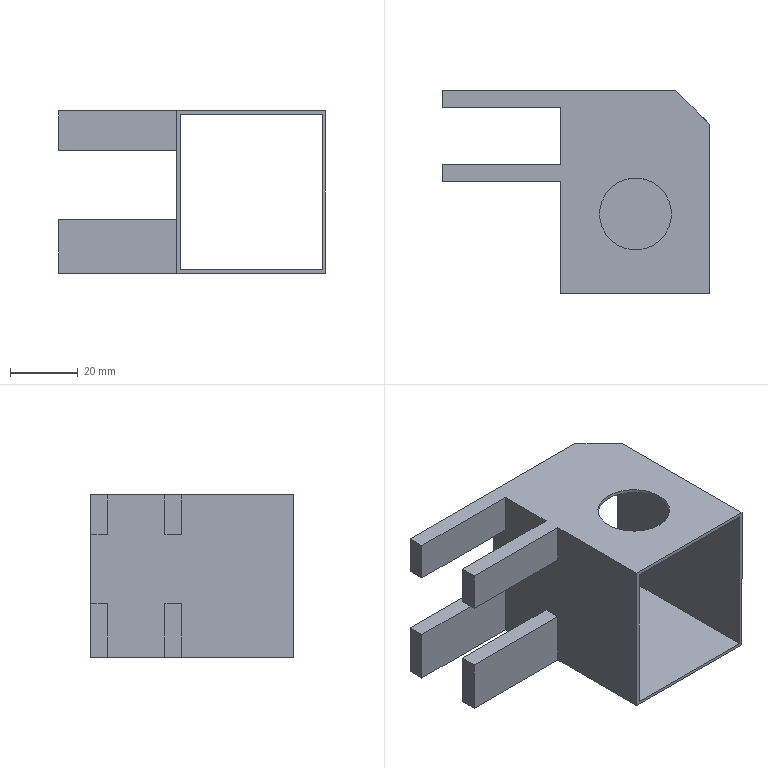Component | SolidWorks | ProtectiveCover-1 | 1 solid | 27 faces | box 79 x 60 x 48 mm | volume 19454 mm3 | plane 25 | cylinder 2 | commonest cylinder face diameters 21.247 x2
STEP:
#1=CARTESIAN_POINT('',(-2.546,-0.8182,36.42));
#2=VERTEX_POINT('',#1);
#3=CARTESIAN_POINT('',(-2.546,-1.655,36.42));
#4=VERTEX_POINT('',#3);
#5=CARTESIAN_POINT('',(-2.546,-1.236,36.42));
#6=DIRECTION('',(-0.,0.,-1.));
#7=DIRECTION('',(0.,-1.,0.));
#8=AXIS2_PLACEMENT_3D('',#5,#6,#7);
#9=CIRCLE('',#8,0.4182);
#10=EDGE_CURVE('',#2,#4,#9,.T.);
#11=ORIENTED_EDGE('',*,*,#10,.T.);
#12=CARTESIAN_POINT('',(-2.546,-1.655,36.459));
#13=VERTEX_POINT('',#12);
#14=CARTESIAN_POINT('',(-2.546,-1.655,35.107));
#15=DIRECTION('',(0.,-0.,1.));
#16=VECTOR('',#15,39.37);
#17=LINE('',#14,#16);
#18=EDGE_CURVE('',#4,#13,#17,.T.);
#19=ORIENTED_EDGE('',*,*,#18,.T.);
#20=CARTESIAN_POINT('',(-2.546,-0.8182,36.459));
#21=VERTEX_POINT('',#20);
#22=CARTESIAN_POINT('',(-2.546,-1.236,36.459));
#23=DIRECTION('',(0.,-0.,1.));
#24=DIRECTION('',(0.,1.,0.));
#25=AXIS2_PLACEMENT_3D('',#22,#23,#24);
#26=CIRCLE('',#25,0.4182);
#27=EDGE_CURVE('',#13,#21,#26,.T.);
#28=ORIENTED_EDGE('',*,*,#27,.T.);
#29=CARTESIAN_POINT('',(-2.546,-0.8182,35.107));
#30=DIRECTION('',(0.,-0.,1.));
#31=VECTOR('',#30,39.37);
#32=LINE('',#29,#31);
#33=EDGE_CURVE('',#2,#21,#32,.T.);
#34=ORIENTED_EDGE('',*,*,#33,.F.);
#35=EDGE_LOOP('',(#11,#19,#28,#34));
#36=FACE_OUTER_BOUND('',#35,.T.);
#37=CARTESIAN_POINT('',(-2.546,-1.236,35.107));
#38=DIRECTION('',(0.,-0.,1.));
#39=DIRECTION('',(0.,1.,0.));
#40=AXIS2_PLACEMENT_3D('',#37,#38,#39);
#41=CYLINDRICAL_SURFACE('',#40,0.4182);
#42=ADVANCED_FACE('',(#36),#41,.F.);
#43=CARTESIAN_POINT('',(-3.417,-0.8584,34.569));
#44=VERTEX_POINT('',#43);
#45=CARTESIAN_POINT('',(-3.417,-0.8584,35.189));
#46=VERTEX_POINT('',#45);
#47=CARTESIAN_POINT('',(-3.417,-0.8584,35.189));
#48=DIRECTION('',(0.,-0.,1.));
#49=VECTOR('',#48,39.37);
#50=LINE('',#47,#49);
#51=EDGE_CURVE('',#44,#46,#50,.T.);
#52=ORIENTED_EDGE('',*,*,#51,.F.);
#53=CARTESIAN_POINT('',(-3.417,-2.16,34.569));
#54=VERTEX_POINT('',#53);
#55=CARTESIAN_POINT('',(-3.417,-2.16,34.569));
#56=DIRECTION('',(0.,1.,0.));
#57=VECTOR('',#56,39.37);
#58=LINE('',#55,#57);
#59=EDGE_CURVE('',#54,#44,#58,.T.);
#60=ORIENTED_EDGE('',*,*,#59,.F.);
#61=CARTESIAN_POINT('',(-3.417,-2.16,36.459));
#62=VERTEX_POINT('',#61);
#63=CARTESIAN_POINT('',(-3.417,-2.16,36.459));
#64=DIRECTION('',(-0.,0.,-1.));
#65=VECTOR('',#64,39.37);
#66=LINE('',#63,#65);
#67=EDGE_CURVE('',#62,#54,#66,.T.);
#68=ORIENTED_EDGE('',*,*,#67,.F.);
#69=CARTESIAN_POINT('',(-3.417,-0.8584,36.459));
#70=VERTEX_POINT('',#69);
#71=CARTESIAN_POINT('',(-3.417,-2.16,36.459));
#72=DIRECTION('',(0.,1.,0.));
#73=VECTOR('',#72,39.37);
#74=LINE('',#71,#73);
#75=EDGE_CURVE('',#62,#70,#74,.T.);
#76=ORIENTED_EDGE('',*,*,#75,.T.);
#77=CARTESIAN_POINT('',(-3.417,-0.8584,35.997));
#78=VERTEX_POINT('',#77);
#79=CARTESIAN_POINT('',(-3.417,-0.8584,36.459));
#80=DIRECTION('',(0.,-0.,1.));
#81=VECTOR('',#80,39.37);
#82=LINE('',#79,#81);
#83=EDGE_CURVE('',#78,#70,#82,.T.);
#84=ORIENTED_EDGE('',*,*,#83,.F.);
#85=CARTESIAN_POINT('',(-3.417,-0.663,35.997));
#86=VERTEX_POINT('',#85);
#87=CARTESIAN_POINT('',(-3.417,-0.8584,35.997));
#88=DIRECTION('',(-0.,-1.,-0.));
#89=VECTOR('',#88,39.37);
#90=LINE('',#87,#89);
#91=EDGE_CURVE('',#86,#78,#90,.T.);
#92=ORIENTED_EDGE('',*,*,#91,.F.);
#93=CARTESIAN_POINT('',(-3.417,-0.663,36.459));
#94=VERTEX_POINT('',#93);
#95=CARTESIAN_POINT('',(-3.417,-0.663,36.459));
#96=DIRECTION('',(-0.,0.,-1.));
#97=VECTOR('',#96,39.37);
#98=LINE('',#95,#97);
#99=EDGE_CURVE('',#94,#86,#98,.T.);
#100=ORIENTED_EDGE('',*,*,#99,.F.);
#101=CARTESIAN_POINT('',(-3.417,0.006968,36.459));
#102=VERTEX_POINT('',#101);
#103=CARTESIAN_POINT('',(-3.417,-2.16,36.459));
#104=DIRECTION('',(0.,1.,0.));
#105=VECTOR('',#104,39.37);
#106=LINE('',#103,#105);
#107=EDGE_CURVE('',#94,#102,#106,.T.);
#108=ORIENTED_EDGE('',*,*,#107,.T.);
#109=CARTESIAN_POINT('',(-3.417,0.006968,35.997));
#110=VERTEX_POINT('',#109);
#111=CARTESIAN_POINT('',(-3.417,0.006968,36.459));
#112=DIRECTION('',(0.,-0.,1.));
#113=VECTOR('',#112,39.37);
#114=LINE('',#111,#113);
#115=EDGE_CURVE('',#110,#102,#114,.T.);
#116=ORIENTED_EDGE('',*,*,#115,.F.);
#117=CARTESIAN_POINT('',(-3.417,0.2024,35.997));
#118=VERTEX_POINT('',#117);
#119=CARTESIAN_POINT('',(-3.417,0.006968,35.997));
#120=DIRECTION('',(-0.,-1.,-0.));
#121=VECTOR('',#120,39.37);
#122=LINE('',#119,#121);
#123=EDGE_CURVE('',#118,#110,#122,.T.);
#124=ORIENTED_EDGE('',*,*,#123,.F.);
#125=CARTESIAN_POINT('',(-3.417,0.2024,35.189));
#126=VERTEX_POINT('',#125);
#127=CARTESIAN_POINT('',(-3.417,0.2024,36.459));
#128=DIRECTION('',(-0.,0.,-1.));
#129=VECTOR('',#128,39.37);
#130=LINE('',#127,#129);
#131=EDGE_CURVE('',#118,#126,#130,.T.);
#132=ORIENTED_EDGE('',*,*,#131,.T.);
#133=CARTESIAN_POINT('',(-3.417,0.006968,35.189));
#134=VERTEX_POINT('',#133);
#135=CARTESIAN_POINT('',(-3.417,0.006968,35.189));
#136=DIRECTION('',(0.,1.,0.));
#137=VECTOR('',#136,39.37);
#138=LINE('',#135,#137);
#139=EDGE_CURVE('',#134,#126,#138,.T.);
#140=ORIENTED_EDGE('',*,*,#139,.F.);
#141=CARTESIAN_POINT('',(-3.417,0.006968,34.569));
#142=VERTEX_POINT('',#141);
#143=CARTESIAN_POINT('',(-3.417,0.006968,35.189));
#144=DIRECTION('',(0.,-0.,1.));
#145=VECTOR('',#144,39.37);
#146=LINE('',#143,#145);
#147=EDGE_CURVE('',#142,#134,#146,.T.);
#148=ORIENTED_EDGE('',*,*,#147,.F.);
#149=CARTESIAN_POINT('',(-3.417,-0.663,34.569));
#150=VERTEX_POINT('',#149);
#151=CARTESIAN_POINT('',(-3.417,-2.16,34.569));
#152=DIRECTION('',(0.,1.,0.));
#153=VECTOR('',#152,39.37);
#154=LINE('',#151,#153);
#155=EDGE_CURVE('',#150,#142,#154,.T.);
#156=ORIENTED_EDGE('',*,*,#155,.F.);
#157=CARTESIAN_POINT('',(-3.417,-0.663,35.189));
#158=VERTEX_POINT('',#157);
#159=CARTESIAN_POINT('',(-3.417,-0.663,35.189));
#160=DIRECTION('',(-0.,0.,-1.));
#161=VECTOR('',#160,39.37);
#162=LINE('',#159,#161);
#163=EDGE_CURVE('',#158,#150,#162,.T.);
#164=ORIENTED_EDGE('',*,*,#163,.F.);
#165=CARTESIAN_POINT('',(-3.417,-0.8584,35.189));
#166=DIRECTION('',(0.,1.,0.));
#167=VECTOR('',#166,39.37);
#168=LINE('',#165,#167);
#169=EDGE_CURVE('',#46,#158,#168,.T.);
#170=ORIENTED_EDGE('',*,*,#169,.F.);
#171=EDGE_LOOP('',(#52,#60,#68,#76,#84,#92,#100,#108,#116,#124,#132,#140,#148,#156,#164,#170));
#172=FACE_OUTER_BOUND('',#171,.T.);
#173=CARTESIAN_POINT('',(-3.417,-2.16,36.459));
#174=DIRECTION('',(1.,-0.,-0.));
#175=DIRECTION('',(-0.,-1.,-0.));
#176=AXIS2_PLACEMENT_3D('',#173,#174,#175);
#177=PLANE('',#176);
#178=ADVANCED_FACE('',(#172),#177,.F.);
#179=CARTESIAN_POINT('',(-1.685,-2.16,36.459));
#180=VERTEX_POINT('',#179);
#181=CARTESIAN_POINT('',(-1.685,-2.16,36.459));
#182=DIRECTION('',(-1.,0.,0.));
#183=VECTOR('',#182,39.37);
#184=LINE('',#181,#183);
#185=EDGE_CURVE('',#180,#62,#184,.T.);
#186=ORIENTED_EDGE('',*,*,#185,.T.);
#187=ORIENTED_EDGE('',*,*,#67,.T.);
#188=CARTESIAN_POINT('',(-1.685,-2.16,34.569));
#189=VERTEX_POINT('',#188);
#190=CARTESIAN_POINT('',(-1.685,-2.16,34.569));
#191=DIRECTION('',(1.,-0.,-0.));
#192=VECTOR('',#191,39.37);
#193=LINE('',#190,#192);
#194=EDGE_CURVE('',#54,#189,#193,.T.);
#195=ORIENTED_EDGE('',*,*,#194,.T.);
#196=CARTESIAN_POINT('',(-1.685,-2.16,36.459));
#197=DIRECTION('',(0.,-0.,1.));
#198=VECTOR('',#197,39.37);
#199=LINE('',#196,#198);
#200=EDGE_CURVE('',#189,#180,#199,.T.);
#201=ORIENTED_EDGE('',*,*,#200,.T.);
#202=EDGE_LOOP('',(#186,#187,#195,#201));
#203=FACE_OUTER_BOUND('',#202,.T.);
#204=CARTESIAN_POINT('',(-1.724,-2.16,36.42));
#205=VERTEX_POINT('',#204);
#206=CARTESIAN_POINT('',(-3.378,-2.16,36.42));
#207=VERTEX_POINT('',#206);
#208=CARTESIAN_POINT('',(-1.724,-2.16,36.42));
#209=DIRECTION('',(-1.,0.,0.));
#210=VECTOR('',#209,39.37);
#211=LINE('',#208,#210);
#212=EDGE_CURVE('',#205,#207,#211,.T.);
#213=ORIENTED_EDGE('',*,*,#212,.F.);
#214=CARTESIAN_POINT('',(-1.724,-2.16,34.609));
#215=VERTEX_POINT('',#214);
#216=CARTESIAN_POINT('',(-1.724,-2.16,36.42));
#217=DIRECTION('',(0.,-0.,1.));
#218=VECTOR('',#217,39.37);
#219=LINE('',#216,#218);
#220=EDGE_CURVE('',#215,#205,#219,.T.);
#221=ORIENTED_EDGE('',*,*,#220,.F.);
#222=CARTESIAN_POINT('',(-3.378,-2.16,34.609));
#223=VERTEX_POINT('',#222);
#224=CARTESIAN_POINT('',(-1.724,-2.16,34.609));
#225=DIRECTION('',(1.,-0.,-0.));
#226=VECTOR('',#225,39.37);
#227=LINE('',#224,#226);
#228=EDGE_CURVE('',#223,#215,#227,.T.);
#229=ORIENTED_EDGE('',*,*,#228,.F.);
#230=CARTESIAN_POINT('',(-3.378,-2.16,36.42));
#231=DIRECTION('',(-0.,0.,-1.));
#232=VECTOR('',#231,39.37);
#233=LINE('',#230,#232);
#234=EDGE_CURVE('',#207,#223,#233,.T.);
#235=ORIENTED_EDGE('',*,*,#234,.F.);
#236=EDGE_LOOP('',(#213,#221,#229,#235));
#237=FACE_BOUND('',#236,.T.);
#238=CARTESIAN_POINT('',(-0.,-2.16,0.1175));
#239=DIRECTION('',(-0.,-1.,-0.));
#240=DIRECTION('',(-1.,0.,0.));
#241=AXIS2_PLACEMENT_3D('',#238,#239,#240);
#242=PLANE('',#241);
#243=ADVANCED_FACE('',(#203,#237),#242,.T.);
#244=CARTESIAN_POINT('',(-2.078,0.2024,36.459));
#245=VERTEX_POINT('',#244);
#246=CARTESIAN_POINT('',(-4.795,0.2024,36.459));
#247=VERTEX_POINT('',#246);
#248=CARTESIAN_POINT('',(-1.685,0.2024,36.459));
#249=DIRECTION('',(-1.,0.,0.));
#250=VECTOR('',#249,39.37);
#251=LINE('',#248,#250);
#252=EDGE_CURVE('',#245,#247,#251,.T.);
#253=ORIENTED_EDGE('',*,*,#252,.F.);
#254=CARTESIAN_POINT('',(-2.078,0.2024,36.42));
#255=VERTEX_POINT('',#254);
#256=CARTESIAN_POINT('',(-2.078,0.2024,0.1175));
#257=DIRECTION('',(-0.,0.,-1.));
#258=VECTOR('',#257,39.37);
#259=LINE('',#256,#258);
#260=EDGE_CURVE('',#245,#255,#259,.T.);
#261=ORIENTED_EDGE('',*,*,#260,.T.);
#262=CARTESIAN_POINT('',(-3.378,0.2024,36.42));
#263=VERTEX_POINT('',#262);
#264=CARTESIAN_POINT('',(-1.724,0.2024,36.42));
#265=DIRECTION('',(-1.,0.,0.));
#266=VECTOR('',#265,39.37);
#267=LINE('',#264,#266);
#268=EDGE_CURVE('',#255,#263,#267,.T.);
#269=ORIENTED_EDGE('',*,*,#268,.T.);
#270=CARTESIAN_POINT('',(-3.378,0.2024,34.609));
#271=VERTEX_POINT('',#270);
#272=CARTESIAN_POINT('',(-3.378,0.2024,36.42));
#273=DIRECTION('',(-0.,0.,-1.));
#274=VECTOR('',#273,39.37);
#275=LINE('',#272,#274);
#276=EDGE_CURVE('',#263,#271,#275,.T.);
#277=ORIENTED_EDGE('',*,*,#276,.T.);
#278=CARTESIAN_POINT('',(-2.078,0.2024,34.609));
#279=VERTEX_POINT('',#278);
#280=CARTESIAN_POINT('',(-1.724,0.2024,34.609));
#281=DIRECTION('',(1.,-0.,-0.));
#282=VECTOR('',#281,39.37);
#283=LINE('',#280,#282);
#284=EDGE_CURVE('',#271,#279,#283,.T.);
#285=ORIENTED_EDGE('',*,*,#284,.T.);
#286=CARTESIAN_POINT('',(-2.078,0.2024,34.569));
#287=VERTEX_POINT('',#286);
#288=CARTESIAN_POINT('',(-2.078,0.2024,0.1175));
#289=DIRECTION('',(-0.,0.,-1.));
#290=VECTOR('',#289,39.37);
#291=LINE('',#288,#290);
#292=EDGE_CURVE('',#279,#287,#291,.T.);
#293=ORIENTED_EDGE('',*,*,#292,.T.);
#294=CARTESIAN_POINT('',(-4.795,0.2024,34.569));
#295=VERTEX_POINT('',#294);
#296=CARTESIAN_POINT('',(-1.685,0.2024,34.569));
#297=DIRECTION('',(1.,-0.,-0.));
#298=VECTOR('',#297,39.37);
#299=LINE('',#296,#298);
#300=EDGE_CURVE('',#295,#287,#299,.T.);
#301=ORIENTED_EDGE('',*,*,#300,.F.);
#302=CARTESIAN_POINT('',(-4.795,0.2024,35.189));
#303=VERTEX_POINT('',#302);
#304=CARTESIAN_POINT('',(-4.795,0.2024,35.189));
#305=DIRECTION('',(-0.,0.,-1.));
#306=VECTOR('',#305,39.37);
#307=LINE('',#304,#306);
#308=EDGE_CURVE('',#303,#295,#307,.T.);
#309=ORIENTED_EDGE('',*,*,#308,.F.);
#310=CARTESIAN_POINT('',(-4.795,0.2024,35.189));
#311=DIRECTION('',(1.,-0.,-0.));
#312=VECTOR('',#311,39.37);
#313=LINE('',#310,#312);
#314=EDGE_CURVE('',#303,#126,#313,.T.);
#315=ORIENTED_EDGE('',*,*,#314,.T.);
#316=ORIENTED_EDGE('',*,*,#131,.F.);
#317=CARTESIAN_POINT('',(-4.795,0.2024,35.997));
#318=VERTEX_POINT('',#317);
#319=CARTESIAN_POINT('',(-4.795,0.2024,35.997));
#320=DIRECTION('',(1.,-0.,-0.));
#321=VECTOR('',#320,39.37);
#322=LINE('',#319,#321);
#323=EDGE_CURVE('',#318,#118,#322,.T.);
#324=ORIENTED_EDGE('',*,*,#323,.F.);
#325=CARTESIAN_POINT('',(-4.795,0.2024,36.459));
#326=DIRECTION('',(-0.,0.,-1.));
#327=VECTOR('',#326,39.37);
#328=LINE('',#325,#327);
#329=EDGE_CURVE('',#247,#318,#328,.T.);
#330=ORIENTED_EDGE('',*,*,#329,.F.);
#331=EDGE_LOOP('',(#253,#261,#269,#277,#285,#293,#301,#309,#315,#316,#324,#330));
#332=FACE_OUTER_BOUND('',#331,.T.);
#333=CARTESIAN_POINT('',(-0.,0.2024,0.1175));
#334=DIRECTION('',(-0.,-1.,-0.));
#335=DIRECTION('',(-1.,0.,0.));
#336=AXIS2_PLACEMENT_3D('',#333,#334,#335);
#337=PLANE('',#336);
#338=ADVANCED_FACE('',(#332),#337,.F.);
#339=CARTESIAN_POINT('',(-2.546,-1.236,36.459));
#340=DIRECTION('',(0.,-0.,1.));
#341=DIRECTION('',(0.,1.,0.));
#342=AXIS2_PLACEMENT_3D('',#339,#340,#341);
#343=CIRCLE('',#342,0.4182);
#344=EDGE_CURVE('',#21,#13,#343,.T.);
#345=ORIENTED_EDGE('',*,*,#344,.F.);
#346=ORIENTED_EDGE('',*,*,#27,.F.);
#347=EDGE_LOOP('',(#345,#346));
#348=FACE_BOUND('',#347,.T.);
#349=CARTESIAN_POINT('',(-1.685,-0.1913,36.459));
#350=VERTEX_POINT('',#349);
#351=CARTESIAN_POINT('',(-1.685,-2.16,36.459));
#352=DIRECTION('',(0.,1.,0.));
#353=VECTOR('',#352,39.37);
#354=LINE('',#351,#353);
#355=EDGE_CURVE('',#180,#350,#354,.T.);
#356=ORIENTED_EDGE('',*,*,#355,.T.);
#357=CARTESIAN_POINT('',(-1.685,-0.1913,36.459));
#358=DIRECTION('',(-0.7071,0.7071,0.));
#359=VECTOR('',#358,39.37);
#360=LINE('',#357,#359);
#361=EDGE_CURVE('',#350,#245,#360,.T.);
#362=ORIENTED_EDGE('',*,*,#361,.T.);
#363=ORIENTED_EDGE('',*,*,#252,.T.);
#364=CARTESIAN_POINT('',(-4.795,0.006968,36.459));
#365=VERTEX_POINT('',#364);
#366=CARTESIAN_POINT('',(-4.795,0.006968,36.459));
#367=DIRECTION('',(0.,1.,0.));
#368=VECTOR('',#367,39.37);
#369=LINE('',#366,#368);
#370=EDGE_CURVE('',#365,#247,#369,.T.);
#371=ORIENTED_EDGE('',*,*,#370,.F.);
#372=CARTESIAN_POINT('',(-4.795,0.006968,36.459));
#373=DIRECTION('',(1.,-0.,-0.));
#374=VECTOR('',#373,39.37);
#375=LINE('',#372,#374);
#376=EDGE_CURVE('',#365,#102,#375,.T.);
#377=ORIENTED_EDGE('',*,*,#376,.T.);
#378=ORIENTED_EDGE('',*,*,#107,.F.);
#379=CARTESIAN_POINT('',(-4.795,-0.663,36.459));
#380=VERTEX_POINT('',#379);
#381=CARTESIAN_POINT('',(-4.795,-0.663,36.459));
#382=DIRECTION('',(1.,-0.,-0.));
#383=VECTOR('',#382,39.37);
#384=LINE('',#381,#383);
#385=EDGE_CURVE('',#380,#94,#384,.T.);
#386=ORIENTED_EDGE('',*,*,#385,.F.);
#387=CARTESIAN_POINT('',(-4.795,-0.8584,36.459));
#388=VERTEX_POINT('',#387);
#389=CARTESIAN_POINT('',(-4.795,-0.8584,36.459));
#390=DIRECTION('',(0.,1.,0.));
#391=VECTOR('',#390,39.37);
#392=LINE('',#389,#391);
#393=EDGE_CURVE('',#388,#380,#392,.T.);
#394=ORIENTED_EDGE('',*,*,#393,.F.);
#395=CARTESIAN_POINT('',(-4.795,-0.8584,36.459));
#396=DIRECTION('',(1.,-0.,-0.));
#397=VECTOR('',#396,39.37);
#398=LINE('',#395,#397);
#399=EDGE_CURVE('',#388,#70,#398,.T.);
#400=ORIENTED_EDGE('',*,*,#399,.T.);
#401=ORIENTED_EDGE('',*,*,#75,.F.);
#402=ORIENTED_EDGE('',*,*,#185,.F.);
#403=EDGE_LOOP('',(#356,#362,#363,#371,#377,#378,#386,#394,#400,#401,#402));
#404=FACE_OUTER_BOUND('',#403,.T.);
#405=CARTESIAN_POINT('',(-1.685,-2.16,36.459));
#406=DIRECTION('',(-0.,0.,-1.));
#407=DIRECTION('',(-0.,-1.,-0.));
#408=AXIS2_PLACEMENT_3D('',#405,#406,#407);
#409=PLANE('',#408);
#410=ADVANCED_FACE('',(#348,#404),#409,.F.);
#411=ORIENTED_EDGE('',*,*,#300,.T.);
#412=CARTESIAN_POINT('',(-1.685,-0.1913,34.569));
#413=VERTEX_POINT('',#412);
#414=CARTESIAN_POINT('',(-1.685,-0.1913,34.569));
#415=DIRECTION('',(0.7071,-0.7071,-0.));
#416=VECTOR('',#415,39.37);
#417=LINE('',#414,#416);
#418=EDGE_CURVE('',#287,#413,#417,.T.);
#419=ORIENTED_EDGE('',*,*,#418,.T.);
#420=CARTESIAN_POINT('',(-1.685,-2.16,34.569));
#421=DIRECTION('',(0.,1.,0.));
#422=VECTOR('',#421,39.37);
#423=LINE('',#420,#422);
#424=EDGE_CURVE('',#189,#413,#423,.T.);
#425=ORIENTED_EDGE('',*,*,#424,.F.);
#426=ORIENTED_EDGE('',*,*,#194,.F.);
#427=ORIENTED_EDGE('',*,*,#59,.T.);
#428=CARTESIAN_POINT('',(-4.795,-0.8584,34.569));
#429=VERTEX_POINT('',#428);
#430=CARTESIAN_POINT('',(-4.795,-0.8584,34.569));
#431=DIRECTION('',(1.,-0.,-0.));
#432=VECTOR('',#431,39.37);
#433=LINE('',#430,#432);
#434=EDGE_CURVE('',#429,#44,#433,.T.);
#435=ORIENTED_EDGE('',*,*,#434,.F.);
#436=CARTESIAN_POINT('',(-4.795,-0.663,34.569));
#437=VERTEX_POINT('',#436);
#438=CARTESIAN_POINT('',(-4.795,-0.8584,34.569));
#439=DIRECTION('',(-0.,-1.,-0.));
#440=VECTOR('',#439,39.37);
#441=LINE('',#438,#440);
#442=EDGE_CURVE('',#437,#429,#441,.T.);
#443=ORIENTED_EDGE('',*,*,#442,.F.);
#444=CARTESIAN_POINT('',(-4.795,-0.663,34.569));
#445=DIRECTION('',(1.,-0.,-0.));
#446=VECTOR('',#445,39.37);
#447=LINE('',#444,#446);
#448=EDGE_CURVE('',#437,#150,#447,.T.);
#449=ORIENTED_EDGE('',*,*,#448,.T.);
#450=ORIENTED_EDGE('',*,*,#155,.T.);
#451=CARTESIAN_POINT('',(-4.795,0.006968,34.569));
#452=VERTEX_POINT('',#451);
#453=CARTESIAN_POINT('',(-4.795,0.006968,34.569));
#454=DIRECTION('',(1.,-0.,-0.));
#455=VECTOR('',#454,39.37);
#456=LINE('',#453,#455);
#457=EDGE_CURVE('',#452,#142,#456,.T.);
#458=ORIENTED_EDGE('',*,*,#457,.F.);
#459=CARTESIAN_POINT('',(-4.795,0.006968,34.569));
#460=DIRECTION('',(-0.,-1.,-0.));
#461=VECTOR('',#460,39.37);
#462=LINE('',#459,#461);
#463=EDGE_CURVE('',#295,#452,#462,.T.);
#464=ORIENTED_EDGE('',*,*,#463,.F.);
#465=EDGE_LOOP('',(#411,#419,#425,#426,#427,#435,#443,#449,#450,#458,#464));
#466=FACE_OUTER_BOUND('',#465,.T.);
#467=CARTESIAN_POINT('',(-1.685,-2.16,34.569));
#468=DIRECTION('',(0.,-0.,1.));
#469=DIRECTION('',(0.,1.,0.));
#470=AXIS2_PLACEMENT_3D('',#467,#468,#469);
#471=PLANE('',#470);
#472=ADVANCED_FACE('',(#466),#471,.F.);
#473=ORIENTED_EDGE('',*,*,#424,.T.);
#474=CARTESIAN_POINT('',(-1.685,-0.1913,36.459));
#475=DIRECTION('',(0.,-0.,1.));
#476=VECTOR('',#475,39.37);
#477=LINE('',#474,#476);
#478=EDGE_CURVE('',#413,#350,#477,.T.);
#479=ORIENTED_EDGE('',*,*,#478,.T.);
#480=ORIENTED_EDGE('',*,*,#355,.F.);
#481=ORIENTED_EDGE('',*,*,#200,.F.);
#482=EDGE_LOOP('',(#473,#479,#480,#481));
#483=FACE_OUTER_BOUND('',#482,.T.);
#484=CARTESIAN_POINT('',(-1.685,-2.16,36.459));
#485=DIRECTION('',(-1.,0.,0.));
#486=DIRECTION('',(0.,1.,0.));
#487=AXIS2_PLACEMENT_3D('',#484,#485,#486);
#488=PLANE('',#487);
#489=ADVANCED_FACE('',(#483),#488,.F.);
#490=CARTESIAN_POINT('',(-1.724,-0.1519,36.42));
#491=VERTEX_POINT('',#490);
#492=CARTESIAN_POINT('',(-1.724,-2.16,36.42));
#493=DIRECTION('',(0.,1.,0.));
#494=VECTOR('',#493,39.37);
#495=LINE('',#492,#494);
#496=EDGE_CURVE('',#205,#491,#495,.T.);
#497=ORIENTED_EDGE('',*,*,#496,.T.);
#498=CARTESIAN_POINT('',(-1.724,-0.1519,34.609));
#499=VERTEX_POINT('',#498);
#500=CARTESIAN_POINT('',(-1.724,-0.1519,36.42));
#501=DIRECTION('',(-0.,0.,-1.));
#502=VECTOR('',#501,39.37);
#503=LINE('',#500,#502);
#504=EDGE_CURVE('',#491,#499,#503,.T.);
#505=ORIENTED_EDGE('',*,*,#504,.T.);
#506=CARTESIAN_POINT('',(-1.724,-2.16,34.609));
#507=DIRECTION('',(0.,1.,0.));
#508=VECTOR('',#507,39.37);
#509=LINE('',#506,#508);
#510=EDGE_CURVE('',#215,#499,#509,.T.);
#511=ORIENTED_EDGE('',*,*,#510,.F.);
#512=ORIENTED_EDGE('',*,*,#220,.T.);
#513=EDGE_LOOP('',(#497,#505,#511,#512));
#514=FACE_OUTER_BOUND('',#513,.T.);
#515=CARTESIAN_POINT('',(-1.724,-2.16,36.42));
#516=DIRECTION('',(-1.,0.,0.));
#517=DIRECTION('',(0.,1.,0.));
#518=AXIS2_PLACEMENT_3D('',#515,#516,#517);
#519=PLANE('',#518);
#520=ADVANCED_FACE('',(#514),#519,.T.);
#521=ORIENTED_EDGE('',*,*,#10,.F.);
#522=CARTESIAN_POINT('',(-2.546,-1.236,36.42));
#523=DIRECTION('',(-0.,0.,-1.));
#524=DIRECTION('',(0.,-1.,0.));
#525=AXIS2_PLACEMENT_3D('',#522,#523,#524);
#526=CIRCLE('',#525,0.4182);
#527=EDGE_CURVE('',#4,#2,#526,.T.);
#528=ORIENTED_EDGE('',*,*,#527,.F.);
#529=EDGE_LOOP('',(#521,#528));
#530=FACE_BOUND('',#529,.T.);
#531=ORIENTED_EDGE('',*,*,#268,.F.);
#532=CARTESIAN_POINT('',(-0.7202,-1.156,36.42));
#533=DIRECTION('',(0.7071,-0.7071,-0.));
#534=VECTOR('',#533,39.37);
#535=LINE('',#532,#534);
#536=EDGE_CURVE('',#255,#491,#535,.T.);
#537=ORIENTED_EDGE('',*,*,#536,.T.);
#538=ORIENTED_EDGE('',*,*,#496,.F.);
#539=ORIENTED_EDGE('',*,*,#212,.T.);
#540=CARTESIAN_POINT('',(-3.378,-2.16,36.42));
#541=DIRECTION('',(0.,1.,0.));
#542=VECTOR('',#541,39.37);
#543=LINE('',#540,#542);
#544=EDGE_CURVE('',#207,#263,#543,.T.);
#545=ORIENTED_EDGE('',*,*,#544,.T.);
#546=EDGE_LOOP('',(#531,#537,#538,#539,#545));
#547=FACE_OUTER_BOUND('',#546,.T.);
#548=CARTESIAN_POINT('',(-1.724,-2.16,36.42));
#549=DIRECTION('',(-0.,0.,-1.));
#550=DIRECTION('',(-0.,-1.,-0.));
#551=AXIS2_PLACEMENT_3D('',#548,#549,#550);
#552=PLANE('',#551);
#553=ADVANCED_FACE('',(#530,#547),#552,.T.);
#554=ORIENTED_EDGE('',*,*,#276,.F.);
#555=ORIENTED_EDGE('',*,*,#544,.F.);
#556=ORIENTED_EDGE('',*,*,#234,.T.);
#557=CARTESIAN_POINT('',(-3.378,-2.16,34.609));
#558=DIRECTION('',(0.,1.,0.));
#559=VECTOR('',#558,39.37);
#560=LINE('',#557,#559);
#561=EDGE_CURVE('',#223,#271,#560,.T.);
#562=ORIENTED_EDGE('',*,*,#561,.T.);
#563=EDGE_LOOP('',(#554,#555,#556,#562));
#564=FACE_OUTER_BOUND('',#563,.T.);
#565=CARTESIAN_POINT('',(-3.378,-2.16,36.42));
#566=DIRECTION('',(1.,-0.,-0.));
#567=DIRECTION('',(-0.,-1.,-0.));
#568=AXIS2_PLACEMENT_3D('',#565,#566,#567);
#569=PLANE('',#568);
#570=ADVANCED_FACE('',(#564),#569,.T.);
#571=ORIENTED_EDGE('',*,*,#510,.T.);
#572=CARTESIAN_POINT('',(-0.7202,-1.156,34.609));
#573=DIRECTION('',(-0.7071,0.7071,0.));
#574=VECTOR('',#573,39.37);
#575=LINE('',#572,#574);
#576=EDGE_CURVE('',#499,#279,#575,.T.);
#577=ORIENTED_EDGE('',*,*,#576,.T.);
#578=ORIENTED_EDGE('',*,*,#284,.F.);
#579=ORIENTED_EDGE('',*,*,#561,.F.);
#580=ORIENTED_EDGE('',*,*,#228,.T.);
#581=EDGE_LOOP('',(#571,#577,#578,#579,#580));
#582=FACE_OUTER_BOUND('',#581,.T.);
#583=CARTESIAN_POINT('',(-1.724,-2.16,34.609));
#584=DIRECTION('',(0.,-0.,1.));
#585=DIRECTION('',(0.,1.,0.));
#586=AXIS2_PLACEMENT_3D('',#583,#584,#585);
#587=PLANE('',#586);
#588=ADVANCED_FACE('',(#582),#587,.T.);
#589=ORIENTED_EDGE('',*,*,#115,.T.);
#590=ORIENTED_EDGE('',*,*,#376,.F.);
#591=CARTESIAN_POINT('',(-4.795,0.006968,35.997));
#592=VERTEX_POINT('',#591);
#593=CARTESIAN_POINT('',(-4.795,0.006968,36.459));
#594=DIRECTION('',(0.,-0.,1.));
#595=VECTOR('',#594,39.37);
#596=LINE('',#593,#595);
#597=EDGE_CURVE('',#592,#365,#596,.T.);
#598=ORIENTED_EDGE('',*,*,#597,.F.);
#599=CARTESIAN_POINT('',(-4.795,0.006968,35.997));
#600=DIRECTION('',(1.,-0.,-0.));
#601=VECTOR('',#600,39.37);
#602=LINE('',#599,#601);
#603=EDGE_CURVE('',#592,#110,#602,.T.);
#604=ORIENTED_EDGE('',*,*,#603,.T.);
#605=EDGE_LOOP('',(#589,#590,#598,#604));
#606=FACE_OUTER_BOUND('',#605,.T.);
#607=CARTESIAN_POINT('',(-4.795,0.006968,36.459));
#608=DIRECTION('',(0.,1.,0.));
#609=DIRECTION('',(1.,-0.,-0.));
#610=AXIS2_PLACEMENT_3D('',#607,#608,#609);
#611=PLANE('',#610);
#612=ADVANCED_FACE('',(#606),#611,.F.);
#613=ORIENTED_EDGE('',*,*,#123,.T.);
#614=ORIENTED_EDGE('',*,*,#603,.F.);
#615=CARTESIAN_POINT('',(-4.795,0.006968,35.997));
#616=DIRECTION('',(-0.,-1.,-0.));
#617=VECTOR('',#616,39.37);
#618=LINE('',#615,#617);
#619=EDGE_CURVE('',#318,#592,#618,.T.);
#620=ORIENTED_EDGE('',*,*,#619,.F.);
#621=ORIENTED_EDGE('',*,*,#323,.T.);
#622=EDGE_LOOP('',(#613,#614,#620,#621));
#623=FACE_OUTER_BOUND('',#622,.T.);
#624=CARTESIAN_POINT('',(-4.795,0.006968,35.997));
#625=DIRECTION('',(0.,-0.,1.));
#626=DIRECTION('',(0.,1.,0.));
#627=AXIS2_PLACEMENT_3D('',#624,#625,#626);
#628=PLANE('',#627);
#629=ADVANCED_FACE('',(#623),#628,.F.);
#630=ORIENTED_EDGE('',*,*,#597,.T.);
#631=ORIENTED_EDGE('',*,*,#370,.T.);
#632=ORIENTED_EDGE('',*,*,#329,.T.);
#633=ORIENTED_EDGE('',*,*,#619,.T.);
#634=EDGE_LOOP('',(#630,#631,#632,#633));
#635=FACE_OUTER_BOUND('',#634,.T.);
#636=CARTESIAN_POINT('',(-4.795,0.2024,0.1175));
#637=DIRECTION('',(1.,-0.,-0.));
#638=DIRECTION('',(-0.,-1.,-0.));
#639=AXIS2_PLACEMENT_3D('',#636,#637,#638);
#640=PLANE('',#639);
#641=ADVANCED_FACE('',(#635),#640,.F.);
#642=ORIENTED_EDGE('',*,*,#147,.T.);
#643=CARTESIAN_POINT('',(-4.795,0.006968,35.189));
#644=VERTEX_POINT('',#643);
#645=CARTESIAN_POINT('',(-4.795,0.006968,35.189));
#646=DIRECTION('',(1.,-0.,-0.));
#647=VECTOR('',#646,39.37);
#648=LINE('',#645,#647);
#649=EDGE_CURVE('',#644,#134,#648,.T.);
#650=ORIENTED_EDGE('',*,*,#649,.F.);
#651=CARTESIAN_POINT('',(-4.795,0.006968,35.189));
#652=DIRECTION('',(0.,-0.,1.));
#653=VECTOR('',#652,39.37);
#654=LINE('',#651,#653);
#655=EDGE_CURVE('',#452,#644,#654,.T.);
#656=ORIENTED_EDGE('',*,*,#655,.F.);
#657=ORIENTED_EDGE('',*,*,#457,.T.);
#658=EDGE_LOOP('',(#642,#650,#656,#657));
#659=FACE_OUTER_BOUND('',#658,.T.);
#660=CARTESIAN_POINT('',(-4.795,0.006968,35.189));
#661=DIRECTION('',(0.,1.,0.));
#662=DIRECTION('',(1.,-0.,-0.));
#663=AXIS2_PLACEMENT_3D('',#660,#661,#662);
#664=PLANE('',#663);
#665=ADVANCED_FACE('',(#659),#664,.F.);
#666=ORIENTED_EDGE('',*,*,#139,.T.);
#667=ORIENTED_EDGE('',*,*,#314,.F.);
#668=CARTESIAN_POINT('',(-4.795,0.006968,35.189));
#669=DIRECTION('',(0.,1.,0.));
#670=VECTOR('',#669,39.37);
#671=LINE('',#668,#670);
#672=EDGE_CURVE('',#644,#303,#671,.T.);
#673=ORIENTED_EDGE('',*,*,#672,.F.);
#674=ORIENTED_EDGE('',*,*,#649,.T.);
#675=EDGE_LOOP('',(#666,#667,#673,#674));
#676=FACE_OUTER_BOUND('',#675,.T.);
#677=CARTESIAN_POINT('',(-4.795,0.006968,35.189));
#678=DIRECTION('',(-0.,0.,-1.));
#679=DIRECTION('',(-0.,-1.,-0.));
#680=AXIS2_PLACEMENT_3D('',#677,#678,#679);
#681=PLANE('',#680);
#682=ADVANCED_FACE('',(#676),#681,.F.);
#683=ORIENTED_EDGE('',*,*,#655,.T.);
#684=ORIENTED_EDGE('',*,*,#672,.T.);
#685=ORIENTED_EDGE('',*,*,#308,.T.);
#686=ORIENTED_EDGE('',*,*,#463,.T.);
#687=EDGE_LOOP('',(#683,#684,#685,#686));
#688=FACE_OUTER_BOUND('',#687,.T.);
#689=CARTESIAN_POINT('',(-4.795,0.2024,0.1175));
#690=DIRECTION('',(1.,-0.,-0.));
#691=DIRECTION('',(-0.,-1.,-0.));
#692=AXIS2_PLACEMENT_3D('',#689,#690,#691);
#693=PLANE('',#692);
#694=ADVANCED_FACE('',(#688),#693,.F.);
#695=ORIENTED_EDGE('',*,*,#18,.F.);
#696=ORIENTED_EDGE('',*,*,#527,.T.);
#697=ORIENTED_EDGE('',*,*,#33,.T.);
#698=ORIENTED_EDGE('',*,*,#344,.T.);
#699=EDGE_LOOP('',(#695,#696,#697,#698));
#700=FACE_OUTER_BOUND('',#699,.T.);
#701=CARTESIAN_POINT('',(-2.546,-1.236,35.107));
#702=DIRECTION('',(0.,-0.,1.));
#703=DIRECTION('',(0.,1.,0.));
#704=AXIS2_PLACEMENT_3D('',#701,#702,#703);
#705=CYLINDRICAL_SURFACE('',#704,0.4182);
#706=ADVANCED_FACE('',(#700),#705,.F.);
#707=ORIENTED_EDGE('',*,*,#536,.F.);
#708=ORIENTED_EDGE('',*,*,#260,.F.);
#709=ORIENTED_EDGE('',*,*,#361,.F.);
#710=ORIENTED_EDGE('',*,*,#478,.F.);
#711=ORIENTED_EDGE('',*,*,#418,.F.);
#712=ORIENTED_EDGE('',*,*,#292,.F.);
#713=ORIENTED_EDGE('',*,*,#576,.F.);
#714=ORIENTED_EDGE('',*,*,#504,.F.);
#715=EDGE_LOOP('',(#707,#708,#709,#710,#711,#712,#713,#714));
#716=FACE_OUTER_BOUND('',#715,.T.);
#717=CARTESIAN_POINT('',(-1.685,-0.1913,36.459));
#718=DIRECTION('',(-0.7071,-0.7071,0.));
#719=DIRECTION('',(0.,-0.,1.));
#720=AXIS2_PLACEMENT_3D('',#717,#718,#719);
#721=PLANE('',#720);
#722=ADVANCED_FACE('',(#716),#721,.F.);
#723=ORIENTED_EDGE('',*,*,#83,.T.);
#724=ORIENTED_EDGE('',*,*,#399,.F.);
#725=CARTESIAN_POINT('',(-4.795,-0.8584,35.997));
#726=VERTEX_POINT('',#725);
#727=CARTESIAN_POINT('',(-4.795,-0.8584,36.459));
#728=DIRECTION('',(0.,-0.,1.));
#729=VECTOR('',#728,39.37);
#730=LINE('',#727,#729);
#731=EDGE_CURVE('',#726,#388,#730,.T.);
#732=ORIENTED_EDGE('',*,*,#731,.F.);
#733=CARTESIAN_POINT('',(-4.795,-0.8584,35.997));
#734=DIRECTION('',(1.,-0.,-0.));
#735=VECTOR('',#734,39.37);
#736=LINE('',#733,#735);
#737=EDGE_CURVE('',#726,#78,#736,.T.);
#738=ORIENTED_EDGE('',*,*,#737,.T.);
#739=EDGE_LOOP('',(#723,#724,#732,#738));
#740=FACE_OUTER_BOUND('',#739,.T.);
#741=CARTESIAN_POINT('',(-4.795,-0.8584,36.459));
#742=DIRECTION('',(0.,1.,0.));
#743=DIRECTION('',(1.,-0.,-0.));
#744=AXIS2_PLACEMENT_3D('',#741,#742,#743);
#745=PLANE('',#744);
#746=ADVANCED_FACE('',(#740),#745,.F.);
#747=ORIENTED_EDGE('',*,*,#99,.T.);
#748=CARTESIAN_POINT('',(-4.795,-0.663,35.997));
#749=VERTEX_POINT('',#748);
#750=CARTESIAN_POINT('',(-4.795,-0.663,35.997));
#751=DIRECTION('',(1.,-0.,-0.));
#752=VECTOR('',#751,39.37);
#753=LINE('',#750,#752);
#754=EDGE_CURVE('',#749,#86,#753,.T.);
#755=ORIENTED_EDGE('',*,*,#754,.F.);
#756=CARTESIAN_POINT('',(-4.795,-0.663,36.459));
#757=DIRECTION('',(-0.,0.,-1.));
#758=VECTOR('',#757,39.37);
#759=LINE('',#756,#758);
#760=EDGE_CURVE('',#380,#749,#759,.T.);
#761=ORIENTED_EDGE('',*,*,#760,.F.);
#762=ORIENTED_EDGE('',*,*,#385,.T.);
#763=EDGE_LOOP('',(#747,#755,#761,#762));
#764=FACE_OUTER_BOUND('',#763,.T.);
#765=CARTESIAN_POINT('',(-4.795,-0.663,36.459));
#766=DIRECTION('',(-0.,-1.,-0.));
#767=DIRECTION('',(-1.,0.,0.));
#768=AXIS2_PLACEMENT_3D('',#765,#766,#767);
#769=PLANE('',#768);
#770=ADVANCED_FACE('',(#764),#769,.F.);
#771=ORIENTED_EDGE('',*,*,#91,.T.);
#772=ORIENTED_EDGE('',*,*,#737,.F.);
#773=CARTESIAN_POINT('',(-4.795,-0.8584,35.997));
#774=DIRECTION('',(-0.,-1.,-0.));
#775=VECTOR('',#774,39.37);
#776=LINE('',#773,#775);
#777=EDGE_CURVE('',#749,#726,#776,.T.);
#778=ORIENTED_EDGE('',*,*,#777,.F.);
#779=ORIENTED_EDGE('',*,*,#754,.T.);
#780=EDGE_LOOP('',(#771,#772,#778,#779));
#781=FACE_OUTER_BOUND('',#780,.T.);
#782=CARTESIAN_POINT('',(-4.795,-0.8584,35.997));
#783=DIRECTION('',(0.,-0.,1.));
#784=DIRECTION('',(0.,1.,0.));
#785=AXIS2_PLACEMENT_3D('',#782,#783,#784);
#786=PLANE('',#785);
#787=ADVANCED_FACE('',(#781),#786,.F.);
#788=ORIENTED_EDGE('',*,*,#731,.T.);
#789=ORIENTED_EDGE('',*,*,#393,.T.);
#790=ORIENTED_EDGE('',*,*,#760,.T.);
#791=ORIENTED_EDGE('',*,*,#777,.T.);
#792=EDGE_LOOP('',(#788,#789,#790,#791));
#793=FACE_OUTER_BOUND('',#792,.T.);
#794=CARTESIAN_POINT('',(-4.795,-0.663,0.1175));
#795=DIRECTION('',(1.,-0.,-0.));
#796=DIRECTION('',(-0.,-1.,-0.));
#797=AXIS2_PLACEMENT_3D('',#794,#795,#796);
#798=PLANE('',#797);
#799=ADVANCED_FACE('',(#793),#798,.F.);
#800=ORIENTED_EDGE('',*,*,#51,.T.);
#801=CARTESIAN_POINT('',(-4.795,-0.8584,35.189));
#802=VERTEX_POINT('',#801);
#803=CARTESIAN_POINT('',(-4.795,-0.8584,35.189));
#804=DIRECTION('',(1.,-0.,-0.));
#805=VECTOR('',#804,39.37);
#806=LINE('',#803,#805);
#807=EDGE_CURVE('',#802,#46,#806,.T.);
#808=ORIENTED_EDGE('',*,*,#807,.F.);
#809=CARTESIAN_POINT('',(-4.795,-0.8584,35.189));
#810=DIRECTION('',(0.,-0.,1.));
#811=VECTOR('',#810,39.37);
#812=LINE('',#809,#811);
#813=EDGE_CURVE('',#429,#802,#812,.T.);
#814=ORIENTED_EDGE('',*,*,#813,.F.);
#815=ORIENTED_EDGE('',*,*,#434,.T.);
#816=EDGE_LOOP('',(#800,#808,#814,#815));
#817=FACE_OUTER_BOUND('',#816,.T.);
#818=CARTESIAN_POINT('',(-4.795,-0.8584,35.189));
#819=DIRECTION('',(0.,1.,0.));
#820=DIRECTION('',(1.,-0.,-0.));
#821=AXIS2_PLACEMENT_3D('',#818,#819,#820);
#822=PLANE('',#821);
#823=ADVANCED_FACE('',(#817),#822,.F.);
#824=ORIENTED_EDGE('',*,*,#169,.T.);
#825=CARTESIAN_POINT('',(-4.795,-0.663,35.189));
#826=VERTEX_POINT('',#825);
#827=CARTESIAN_POINT('',(-4.795,-0.663,35.189));
#828=DIRECTION('',(1.,-0.,-0.));
#829=VECTOR('',#828,39.37);
#830=LINE('',#827,#829);
#831=EDGE_CURVE('',#826,#158,#830,.T.);
#832=ORIENTED_EDGE('',*,*,#831,.F.);
#833=CARTESIAN_POINT('',(-4.795,-0.8584,35.189));
#834=DIRECTION('',(0.,1.,0.));
#835=VECTOR('',#834,39.37);
#836=LINE('',#833,#835);
#837=EDGE_CURVE('',#802,#826,#836,.T.);
#838=ORIENTED_EDGE('',*,*,#837,.F.);
#839=ORIENTED_EDGE('',*,*,#807,.T.);
#840=EDGE_LOOP('',(#824,#832,#838,#839));
#841=FACE_OUTER_BOUND('',#840,.T.);
#842=CARTESIAN_POINT('',(-4.795,-0.8584,35.189));
#843=DIRECTION('',(-0.,0.,-1.));
#844=DIRECTION('',(-0.,-1.,-0.));
#845=AXIS2_PLACEMENT_3D('',#842,#843,#844);
#846=PLANE('',#845);
#847=ADVANCED_FACE('',(#841),#846,.F.);
#848=ORIENTED_EDGE('',*,*,#163,.T.);
#849=ORIENTED_EDGE('',*,*,#448,.F.);
#850=CARTESIAN_POINT('',(-4.795,-0.663,35.189));
#851=DIRECTION('',(-0.,0.,-1.));
#852=VECTOR('',#851,39.37);
#853=LINE('',#850,#852);
#854=EDGE_CURVE('',#826,#437,#853,.T.);
#855=ORIENTED_EDGE('',*,*,#854,.F.);
#856=ORIENTED_EDGE('',*,*,#831,.T.);
#857=EDGE_LOOP('',(#848,#849,#855,#856));
#858=FACE_OUTER_BOUND('',#857,.T.);
#859=CARTESIAN_POINT('',(-4.795,-0.663,35.189));
#860=DIRECTION('',(-0.,-1.,-0.));
#861=DIRECTION('',(-1.,0.,0.));
#862=AXIS2_PLACEMENT_3D('',#859,#860,#861);
#863=PLANE('',#862);
#864=ADVANCED_FACE('',(#858),#863,.F.);
#865=ORIENTED_EDGE('',*,*,#813,.T.);
#866=ORIENTED_EDGE('',*,*,#837,.T.);
#867=ORIENTED_EDGE('',*,*,#854,.T.);
#868=ORIENTED_EDGE('',*,*,#442,.T.);
#869=EDGE_LOOP('',(#865,#866,#867,#868));
#870=FACE_OUTER_BOUND('',#869,.T.);
#871=CARTESIAN_POINT('',(-4.795,-0.663,0.1175));
#872=DIRECTION('',(1.,-0.,-0.));
#873=DIRECTION('',(-0.,-1.,-0.));
#874=AXIS2_PLACEMENT_3D('',#871,#872,#873);
#875=PLANE('',#874);
#876=ADVANCED_FACE('',(#870),#875,.F.);
#877=CLOSED_SHELL('',(#42,#178,#243,#338,#410,#472,#489,#520,#553,#570,#588,#612,#629,#641,#665,#682,#694,#706,#722,#746,#770,#787,#799,#823,#847,#864,#876));
#878=MANIFOLD_SOLID_BREP('',#877);
#879=CARTESIAN_POINT('',(0.,0.,0.));
#880=DIRECTION('',(0.,0.,1.));
#881=DIRECTION('',(1.,0.,0.));
#882=AXIS2_PLACEMENT_3D('',#879,#880,#881);
#883=(LENGTH_UNIT()NAMED_UNIT(*)SI_UNIT($,.METRE.));
#884=LENGTH_MEASURE_WITH_UNIT(LENGTH_MEASURE(0.0254),#883);
#885=DIMENSIONAL_EXPONENTS(1.,0.,0.,0.,0.,0.,0.);
#886=(CONVERSION_BASED_UNIT('',#884)LENGTH_UNIT()NAMED_UNIT(#885));
#887=UNCERTAINTY_MEASURE_WITH_UNIT(LENGTH_MEASURE(0.00001),#886,'','');
#888=(NAMED_UNIT(*)PLANE_ANGLE_UNIT()SI_UNIT($,.RADIAN.));
#889=(NAMED_UNIT(*)SI_UNIT($,.STERADIAN.)SOLID_ANGLE_UNIT());
#890=(GEOMETRIC_REPRESENTATION_CONTEXT(3)GLOBAL_UNCERTAINTY_ASSIGNED_CONTEXT((#887))GLOBAL_UNIT_ASSIGNED_CONTEXT((#886,#888,#889))REPRESENTATION_CONTEXT('',''));
#891=ADVANCED_BREP_SHAPE_REPRESENTATION('',(#878,#882),#890);
#892=COLOUR_RGB('',0.7922,0.8196,0.9333);
#893=FILL_AREA_STYLE_COLOUR('',#892);
#894=FILL_AREA_STYLE('',(#893));
#895=SURFACE_STYLE_FILL_AREA(#894);
#896=SURFACE_SIDE_STYLE('',(#895));
#897=SURFACE_STYLE_USAGE(.BOTH.,#896);
#898=PRESENTATION_STYLE_ASSIGNMENT((#897));
#899=STYLED_ITEM('',(#898),#878);
#900=(LENGTH_UNIT()NAMED_UNIT(*)SI_UNIT($,.METRE.));
#901=LENGTH_MEASURE_WITH_UNIT(LENGTH_MEASURE(0.0254),#900);
#902=DIMENSIONAL_EXPONENTS(1.,0.,0.,0.,0.,0.,0.);
#903=(CONVERSION_BASED_UNIT('',#901)LENGTH_UNIT()NAMED_UNIT(#902));
#904=UNCERTAINTY_MEASURE_WITH_UNIT(LENGTH_MEASURE(0.00001),#903,'','');
#905=(NAMED_UNIT(*)PLANE_ANGLE_UNIT()SI_UNIT($,.RADIAN.));
#906=(NAMED_UNIT(*)SI_UNIT($,.STERADIAN.)SOLID_ANGLE_UNIT());
#907=(GEOMETRIC_REPRESENTATION_CONTEXT(3)GLOBAL_UNCERTAINTY_ASSIGNED_CONTEXT((#904))GLOBAL_UNIT_ASSIGNED_CONTEXT((#903,#905,#906))REPRESENTATION_CONTEXT('',''));
#908=MECHANICAL_DESIGN_GEOMETRIC_PRESENTATION_REPRESENTATION('',(#899),#907);
#909=PRESENTATION_LAYER_ASSIGNMENT('','',(#899));